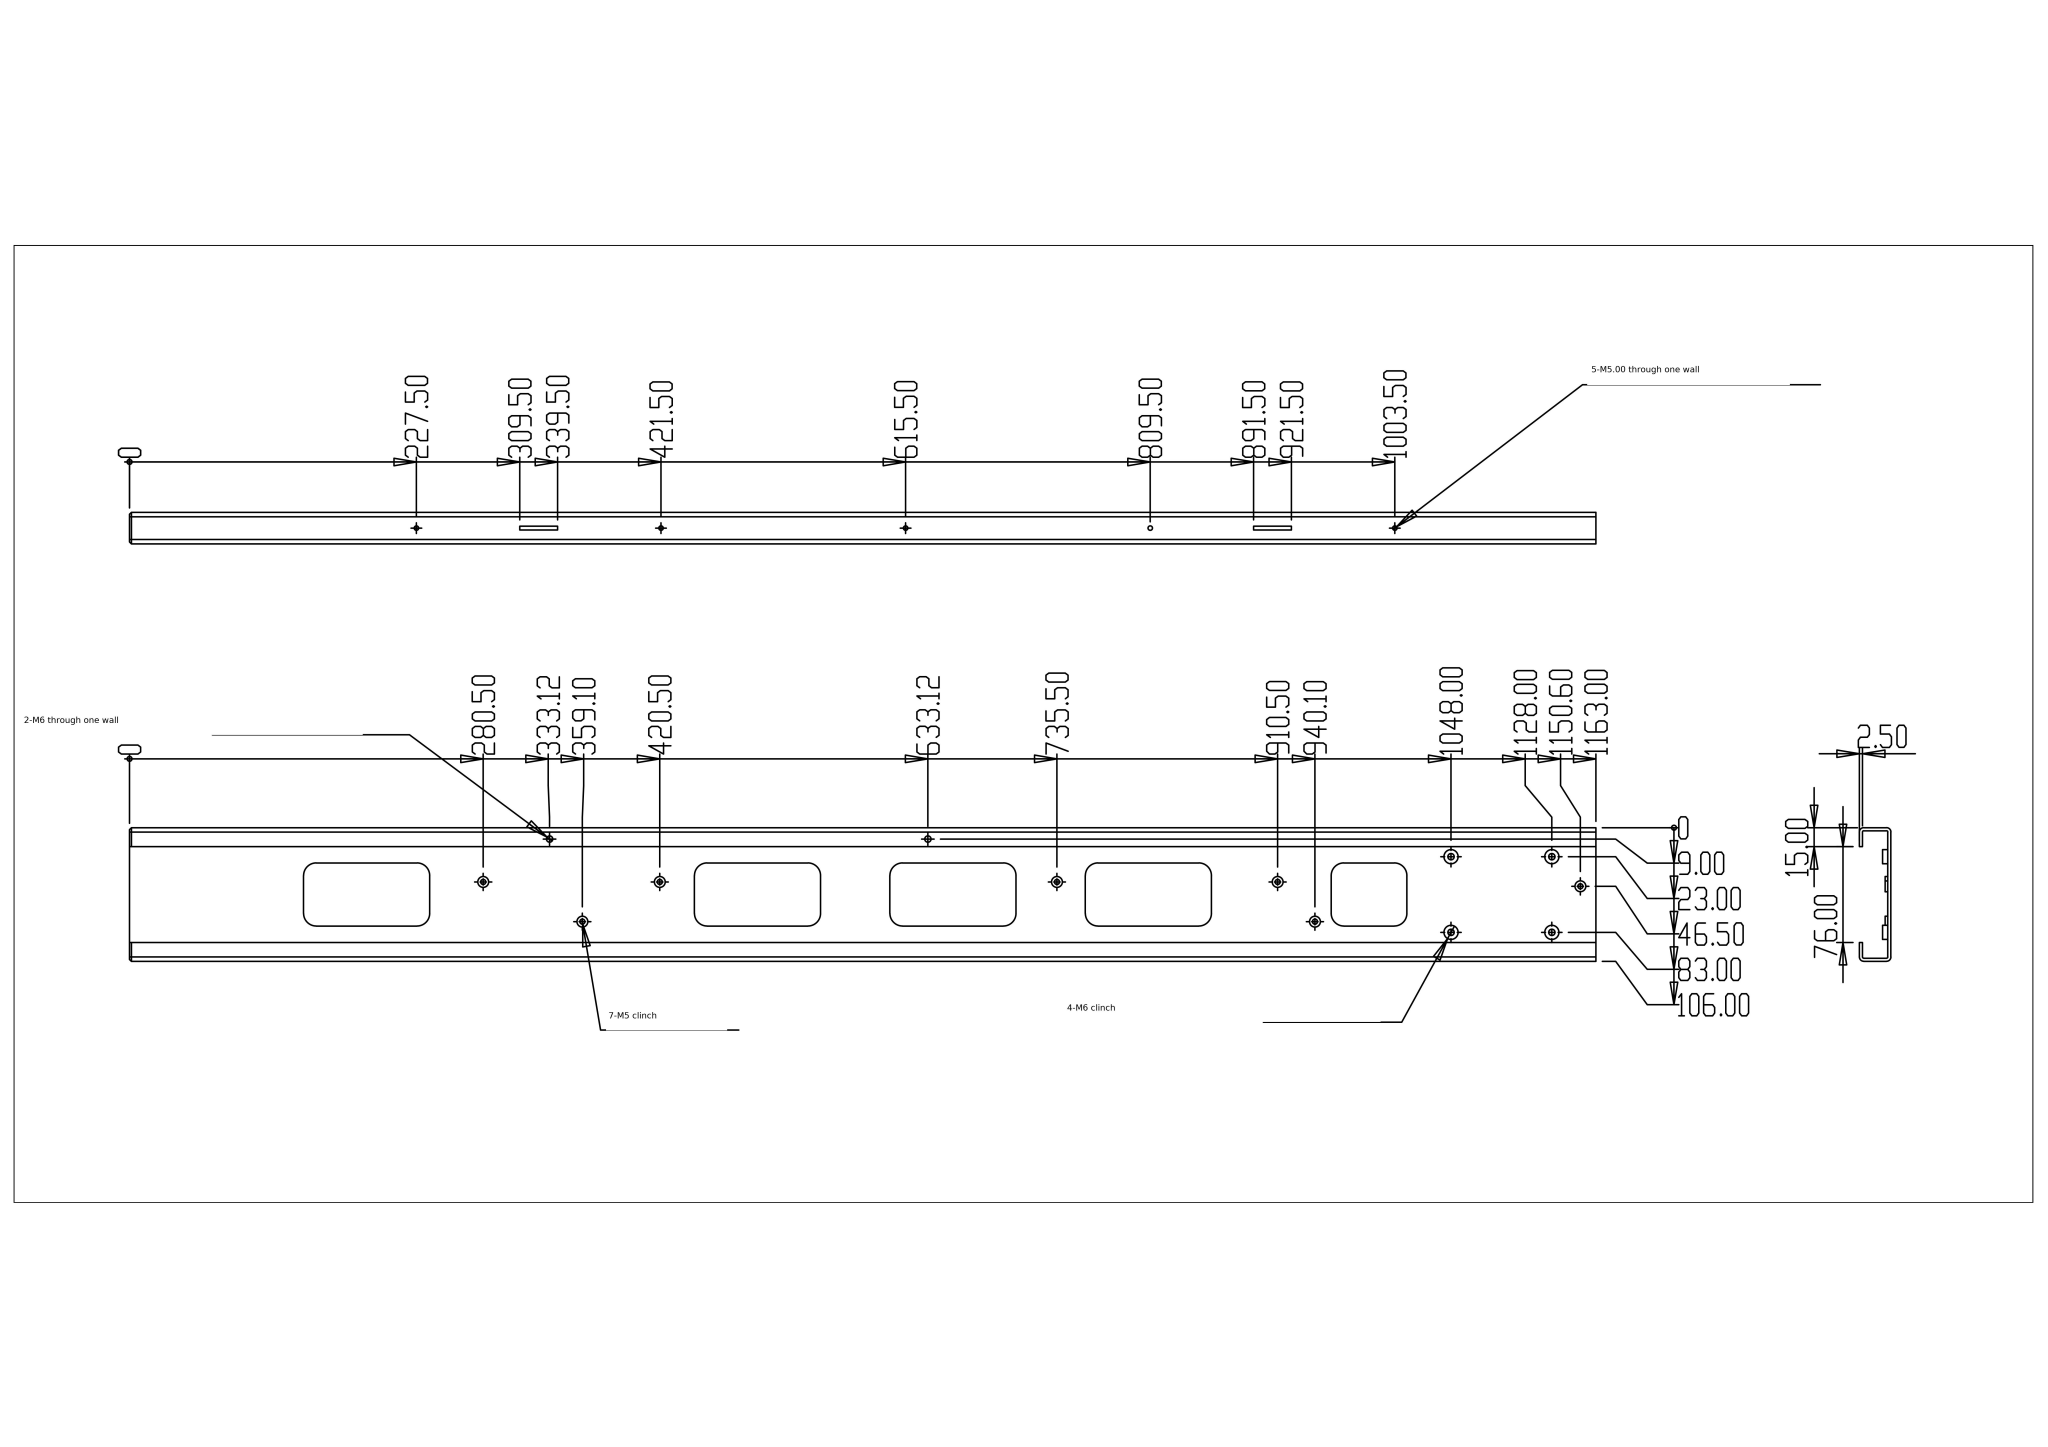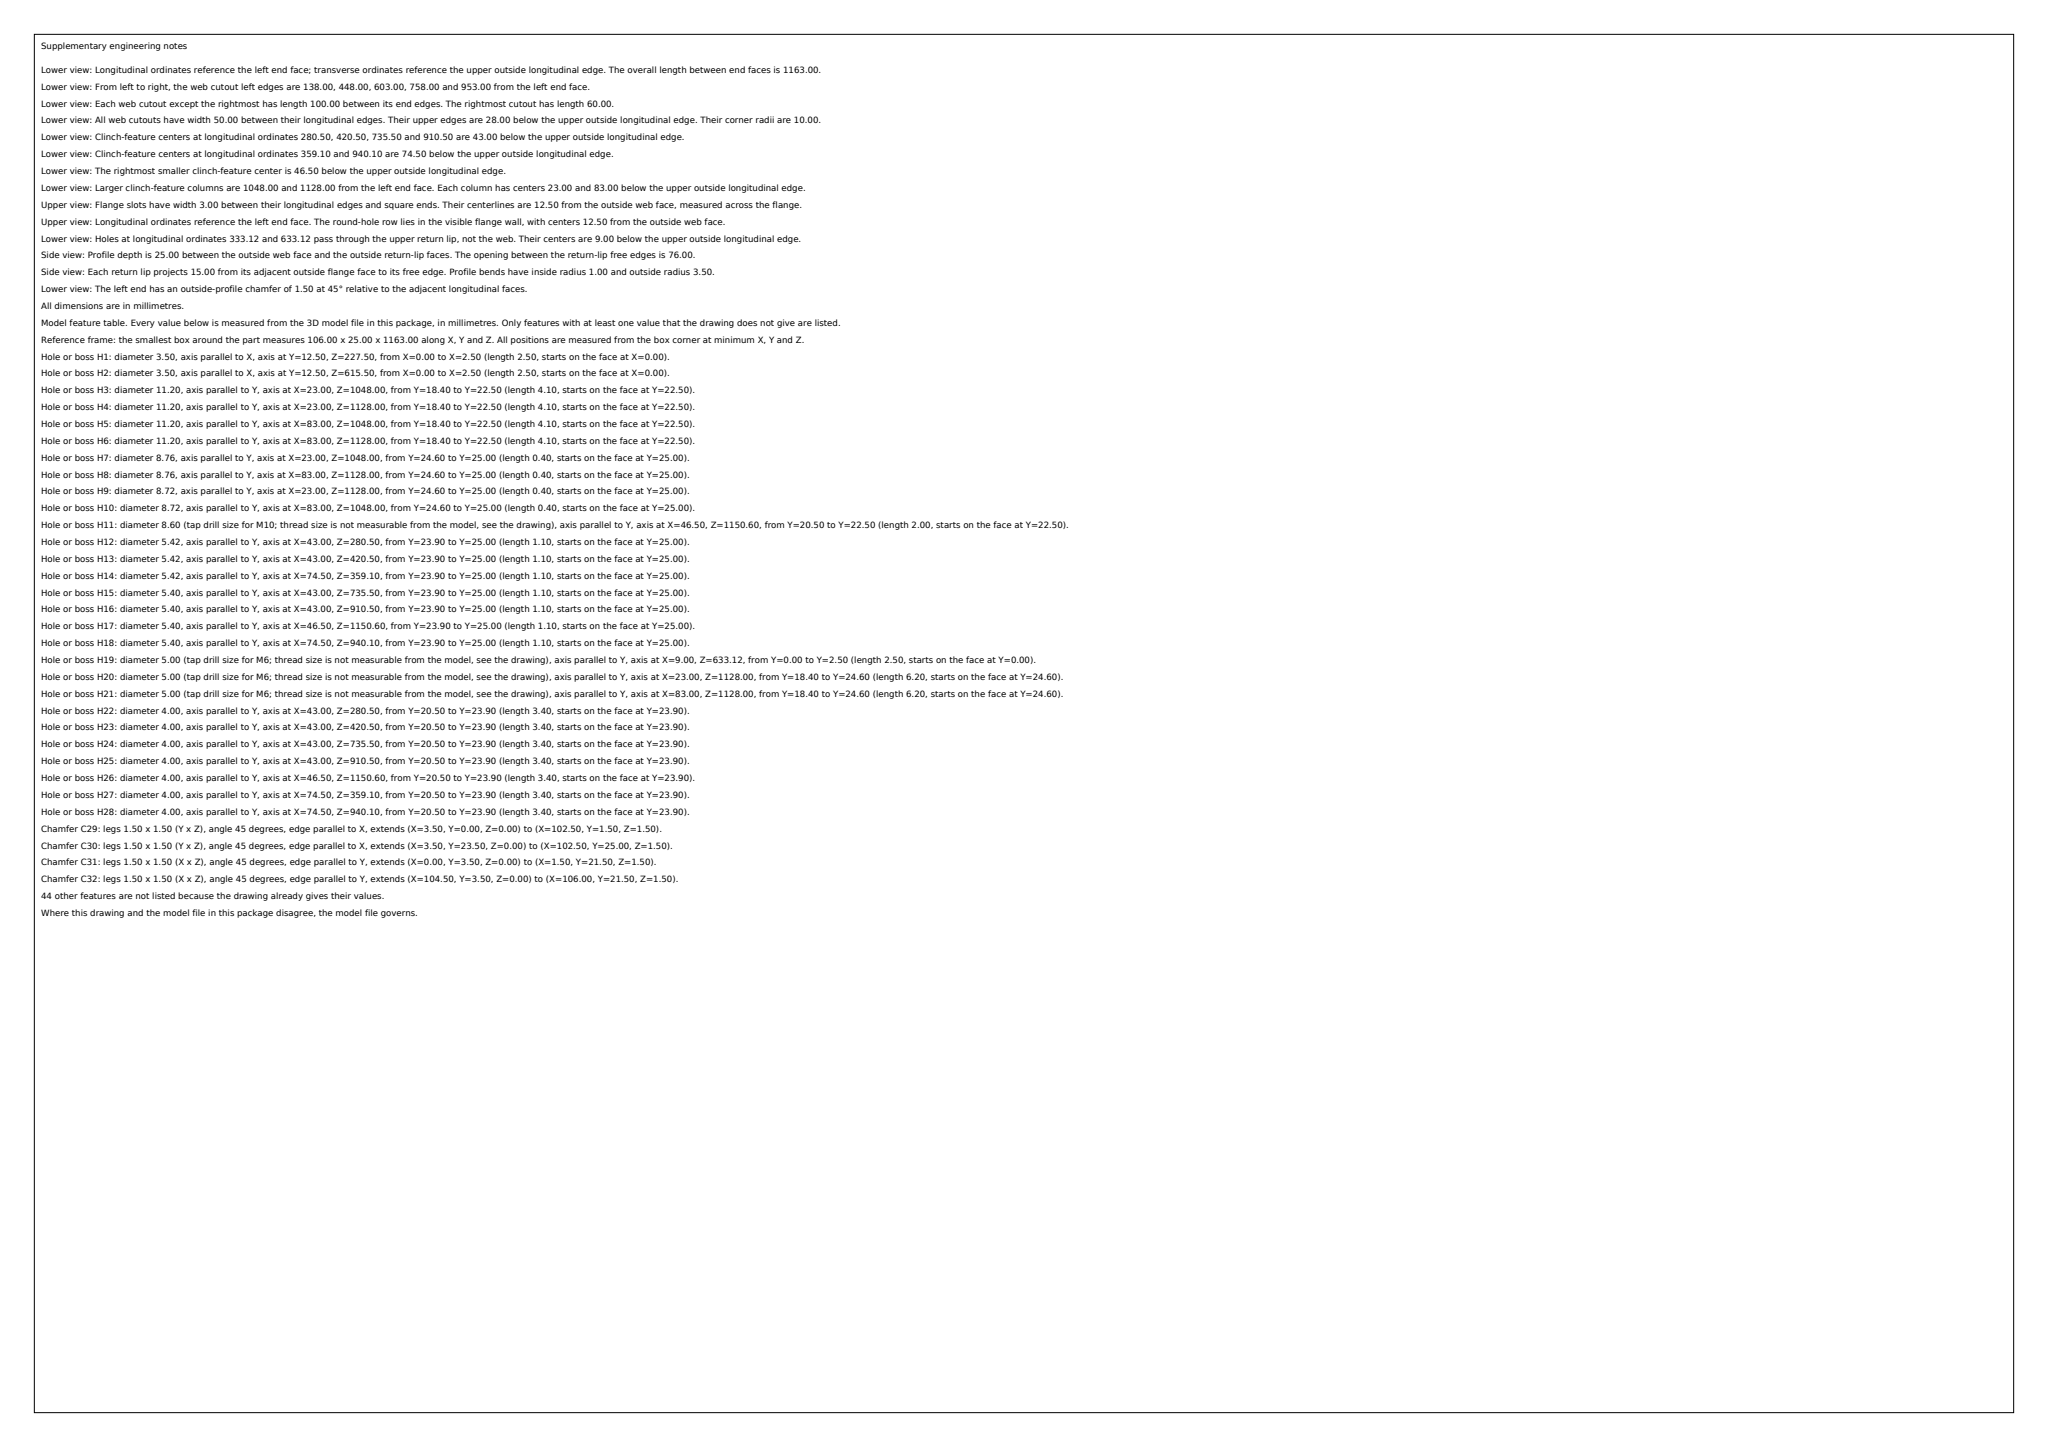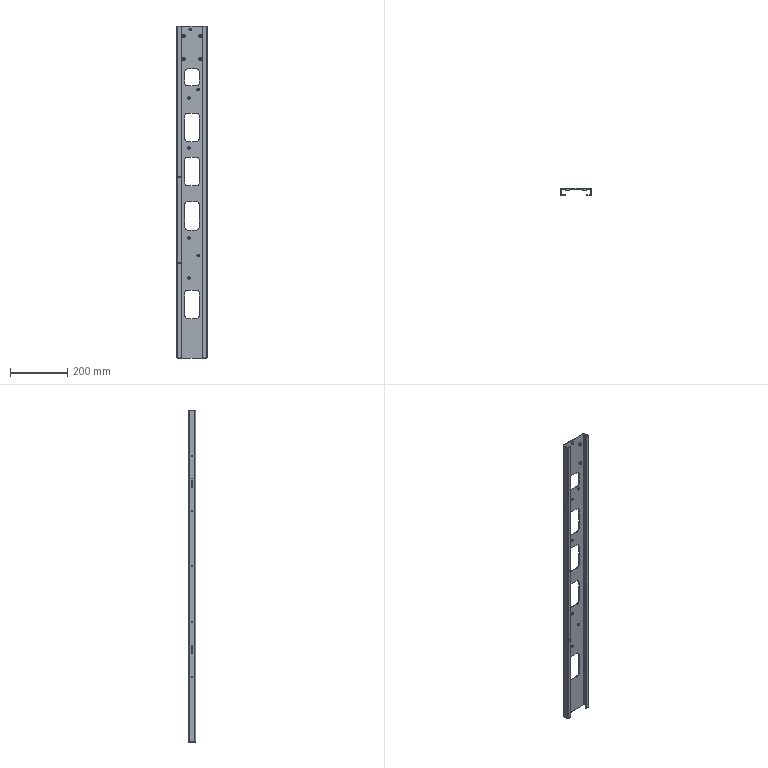Part | SolidWorks | mm | 1 solid | 181 faces | box 106 x 25 x 1163 mm | volume 444564 mm3 | cylinder 108 | plane 69 | cone 4 | commonest cylinder face diameters 20 x20 4 x14 8.6 x14 5.41 x14 5 x12 3.5 x10 11.2 x8 8.75 x4
Drawing notes:
SECTION: OVERALL PROFILE DEPTH 25.00 | from the solid: bbox_xyz y = 25.0; y planes 0.0 and 25.0
ALL ROLL-FORM CORNERS: INNER R1, OUTER R3.5 (4 PL) | from the solid: cylinders Ø2.0 z-axis at (3.5,3.5),(3.5,21.5),(102.5,3.5),(102.5,21.5) L=1163 and Ø7.0 same pos L=1161.5
5 WEB CUTOUTS 50 WIDE x 100 LG (LAST 60 LG), R10 CORNERS | from the solid: x planes 28.0 & 78.0 (5 ea); z pairs 138/238,448/548,603/703,758/858,953/1013; Ø20 y-axis end cyls
WEB CUTOUTS AT Z=138,448,603,758,953; X=28.00 TO 78.00 | from the solid: z planes 138,238,448,548,603,703,758,858,953,1013; x planes 28.0/78.0
7-M5 CLINCH ROWS: X=43.00 (4), X=74.50 (2), X=46.50 (1) | from the solid: Ø4.0 y-axis holes at x=43.0 (z 280.5,420.5,735.5,910.5), x=74.5 (z 359.1,940.1), x=46.5 (z 1150.6)
SIDE WALL SLOTS 30 LG x 3.00 WIDE, Y=11.00 TO 14.00 | from the solid: z planes 309.5/339.5 & 891.5/921.5; y planes 11.0 (2) and 14.0 (2)
5-M5 THRU ONE WALL ON Y=12.50 CL | from the solid: Ø3.5 x-axis holes at y=12.5, z=227.5,421.5,615.5,809.5,1003.5
SIDE HOLES: 4 PL CSK 90° x Ø7.0; HOLE AT 809.50 PLAIN Ø3.5 | from the solid: cones [90.0, 7.0, 4]; five Ø3.5 x-axis holes
build123d program:
from build123d import *

# Parameters (mm, degrees)
BOSS_EXTRUDE1_DEPTH      = 1163
CHAMFER1_SIZE            = 1.5
CUT_EXTRUDE1_REACH       = 1168.823
CUT_EXTRUDE2_REACH       = 1170.088
SKETCH3_R                = 1.75
SKETCH3_W                = 30
SKETCH3_H                = 3
BOSS_EXTRUDE2_DEPTH      = 2
BOSS_EXTRUDE2_DEPTH_BACK = 1.4
SKETCH4_R                = 4.3
SKETCH4_R_2              = 2
BOSS_EXTRUDE3_DEPTH      = 4.1
BOSS_EXTRUDE3_DEPTH_BACK = 2.1
SKETCH5_R                = 5.6
SKETCH5_R_2              = 2.5
CUT_EXTRUDE3_REACH       = 1168.823
SKETCH6_R                = 2.5


with BuildPart() as part:
    # Sketch1 → Boss-Extrude1 (new body)
    with BuildSketch(Plane.XY):
        with BuildLine():
            Line((-76, 0), (-76, 2.5))
            Line((-76, 2.5), (-79, 2.5))
            Line((-79, 2.5), (-87.5, 2.5))
            ThreePointArc((-87.5, 2.5), (-88.207, 2.793), (-88.5, 3.5))
            Line((-88.5, 3.5), (-88.5, 21.5))
            ThreePointArc((-88.5, 21.5), (-88.207, 22.207), (-87.5, 22.5))
            Line((-87.5, 22.5), (11.5, 22.5))
            ThreePointArc((11.5, 22.5), (12.207, 22.207), (12.5, 21.5))
            Line((12.5, 21.5), (12.5, 3.5))
            ThreePointArc((12.5, 3.5), (12.207, 2.793), (11.5, 2.5))
            Line((11.5, 2.5), (3, 2.5))
            Line((3, 2.5), (0, 2.5))
            Line((0, 2.5), (0, 0))
            Line((0, 0), (3, 0))
            Line((3, 0), (11.5, 0))
            ThreePointArc((11.5, 0), (13.975, 1.025), (15, 3.5))
            Line((15, 3.5), (15, 21.5))
            ThreePointArc((15, 21.5), (13.975, 23.975), (11.5, 25))
            Line((11.5, 25), (-87.5, 25))
            ThreePointArc((-87.5, 25), (-89.975, 23.975), (-91, 21.5))
            Line((-91, 21.5), (-91, 3.5))
            ThreePointArc((-91, 3.5), (-89.975, 1.025), (-87.5, 0))
            Line((-87.5, 0), (-79, 0))
            Line((-79, 0), (-76, 0))
        make_face()
    extrude(amount=BOSS_EXTRUDE1_DEPTH)

    # Chamfer1
    chamfer1_edges = [part.edges().sort_by_distance(p)[0] for p in [
        (-81.75, 0, 0),
        (-89.975, 1.025, 0),
        (-91, 12.5, 0),
        (-89.975, 23.975, 0),
        (-38, 25, 0),
        (13.975, 23.975, 0),
        (15, 12.5, 0),
        (13.975, 1.025, 0),
        (5.75, 0, 0),
    ]]
    chamfer(chamfer1_edges, length=CHAMFER1_SIZE)

    # Sketch2 → Cut-Extrude1 (cut, up to next)
    with BuildSketch(Plane(origin=(0, 25, 0), x_dir=(1, 0, 0), z_dir=(0, 1, 0)), mode=Mode.PRIVATE) as cut_extrude1_sk1:
        with BuildLine():
            Line((-23, -953), (-53, -953))
            ThreePointArc((-53, -953), (-60.071, -955.929), (-63, -963))
            Line((-63, -963), (-63, -1003))
            ThreePointArc((-63, -1003), (-60.071, -1010.071), (-53, -1013))
            Line((-53, -1013), (-23, -1013))
            ThreePointArc((-23, -1013), (-15.929, -1010.071), (-13, -1003))
            Line((-13, -1003), (-13, -963))
            ThreePointArc((-13, -963), (-15.929, -955.929), (-23, -953))
        make_face()
    cut_extrude1_tool1 = extrude(cut_extrude1_sk1.sketch, amount=-CUT_EXTRUDE1_REACH, mode=Mode.PRIVATE) & part.part
    # Sketch2 → Cut-Extrude1 (cut, up to next)
    with BuildSketch(Plane(origin=(0, 25, 0), x_dir=(1, 0, 0), z_dir=(0, 1, 0)), mode=Mode.PRIVATE) as cut_extrude1_sk2:
        with BuildLine():
            Line((-23, -603), (-53, -603))
            ThreePointArc((-53, -603), (-60.071, -605.929), (-63, -613))
            Line((-63, -613), (-63, -693))
            ThreePointArc((-63, -693), (-60.071, -700.071), (-53, -703))
            Line((-53, -703), (-23, -703))
            ThreePointArc((-23, -703), (-15.929, -700.071), (-13, -693))
            Line((-13, -693), (-13, -613))
            ThreePointArc((-13, -613), (-15.929, -605.929), (-23, -603))
        make_face()
    cut_extrude1_tool2 = extrude(cut_extrude1_sk2.sketch, amount=-CUT_EXTRUDE1_REACH, mode=Mode.PRIVATE) & part.part
    # Sketch2 → Cut-Extrude1 (cut, up to next)
    with BuildSketch(Plane(origin=(0, 25, 0), x_dir=(1, 0, 0), z_dir=(0, 1, 0)), mode=Mode.PRIVATE) as cut_extrude1_sk3:
        with BuildLine():
            Line((-13, -848), (-13, -768))
            ThreePointArc((-13, -768), (-15.929, -760.929), (-23, -758))
            Line((-23, -758), (-53, -758))
            ThreePointArc((-53, -758), (-60.071, -760.929), (-63, -768))
            Line((-63, -768), (-63, -848))
            ThreePointArc((-63, -848), (-60.071, -855.071), (-53, -858))
            Line((-53, -858), (-23, -858))
            ThreePointArc((-23, -858), (-15.929, -855.071), (-13, -848))
        make_face()
    cut_extrude1_tool3 = extrude(cut_extrude1_sk3.sketch, amount=-CUT_EXTRUDE1_REACH, mode=Mode.PRIVATE) & part.part
    # Sketch2 → Cut-Extrude1 (cut, up to next)
    with BuildSketch(Plane(origin=(0, 25, 0), x_dir=(1, 0, 0), z_dir=(0, 1, 0)), mode=Mode.PRIVATE) as cut_extrude1_sk4:
        with BuildLine():
            Line((-53, -548), (-23, -548))
            ThreePointArc((-23, -548), (-15.929, -545.071), (-13, -538))
            Line((-13, -538), (-13, -458))
            ThreePointArc((-13, -458), (-15.929, -450.929), (-23, -448))
            Line((-23, -448), (-53, -448))
            ThreePointArc((-53, -448), (-60.071, -450.929), (-63, -458))
            Line((-63, -458), (-63, -538))
            ThreePointArc((-63, -538), (-60.071, -545.071), (-53, -548))
        make_face()
    cut_extrude1_tool4 = extrude(cut_extrude1_sk4.sketch, amount=-CUT_EXTRUDE1_REACH, mode=Mode.PRIVATE) & part.part
    # Sketch2 → Cut-Extrude1 (cut, up to next)
    with BuildSketch(Plane(origin=(0, 25, 0), x_dir=(1, 0, 0), z_dir=(0, 1, 0)), mode=Mode.PRIVATE) as cut_extrude1_sk5:
        with BuildLine():
            Line((-13, -228), (-13, -148))
            ThreePointArc((-13, -148), (-15.929, -140.929), (-23, -138))
            Line((-23, -138), (-53, -138))
            ThreePointArc((-53, -138), (-60.071, -140.929), (-63, -148))
            Line((-63, -148), (-63, -228))
            ThreePointArc((-63, -228), (-60.071, -235.071), (-53, -238))
            Line((-53, -238), (-23, -238))
            ThreePointArc((-23, -238), (-15.929, -235.071), (-13, -228))
        make_face()
    cut_extrude1_tool5 = extrude(cut_extrude1_sk5.sketch, amount=-CUT_EXTRUDE1_REACH, mode=Mode.PRIVATE) & part.part
    # Sketch2 → Cut-Extrude1 (cut, up to next)
    with BuildSketch(Plane(origin=(0, 25, 0), x_dir=(1, 0, 0), z_dir=(0, 1, 0)), mode=Mode.PRIVATE) as cut_extrude1_sk6:
        with BuildLine():
            ThreePointArc((-41.795, -1150.6), (-44.5, -1147.895), (-47.205, -1150.6))
            ThreePointArc((-47.205, -1150.6), (-44.5, -1153.305), (-41.795, -1150.6))
        make_face()
    cut_extrude1_tool6 = extrude(cut_extrude1_sk6.sketch, amount=-CUT_EXTRUDE1_REACH, mode=Mode.PRIVATE) & part.part
    # Sketch2 → Cut-Extrude1 (cut, up to next)
    with BuildSketch(Plane(origin=(0, 25, 0), x_dir=(1, 0, 0), z_dir=(0, 1, 0)), mode=Mode.PRIVATE) as cut_extrude1_sk7:
        with BuildLine():
            ThreePointArc((-63.635, -1128), (-68, -1123.635), (-72.365, -1128))
            ThreePointArc((-72.365, -1128), (-68, -1132.365), (-63.635, -1128))
        make_face()
    cut_extrude1_tool7 = extrude(cut_extrude1_sk7.sketch, amount=-CUT_EXTRUDE1_REACH, mode=Mode.PRIVATE) & part.part
    # Sketch2 → Cut-Extrude1 (cut, up to next)
    with BuildSketch(Plane(origin=(0, 25, 0), x_dir=(1, 0, 0), z_dir=(0, 1, 0)), mode=Mode.PRIVATE) as cut_extrude1_sk8:
        with BuildLine():
            ThreePointArc((-3.625, -1128), (-8, -1123.625), (-12.375, -1128))
            ThreePointArc((-12.375, -1128), (-8, -1132.375), (-3.625, -1128))
        make_face()
    cut_extrude1_tool8 = extrude(cut_extrude1_sk8.sketch, amount=-CUT_EXTRUDE1_REACH, mode=Mode.PRIVATE) & part.part
    # Sketch2 → Cut-Extrude1 (cut, up to next)
    with BuildSketch(Plane(origin=(0, 25, 0), x_dir=(1, 0, 0), z_dir=(0, 1, 0)), mode=Mode.PRIVATE) as cut_extrude1_sk9:
        with BuildLine():
            ThreePointArc((-3.635, -1048), (-8, -1043.635), (-12.365, -1048))
            ThreePointArc((-12.365, -1048), (-8, -1052.365), (-3.635, -1048))
        make_face()
    cut_extrude1_tool9 = extrude(cut_extrude1_sk9.sketch, amount=-CUT_EXTRUDE1_REACH, mode=Mode.PRIVATE) & part.part
    # Sketch2 → Cut-Extrude1 (cut, up to next)
    with BuildSketch(Plane(origin=(0, 25, 0), x_dir=(1, 0, 0), z_dir=(0, 1, 0)), mode=Mode.PRIVATE) as cut_extrude1_sk10:
        with BuildLine():
            ThreePointArc((-63.625, -1048), (-68, -1043.625), (-72.375, -1048))
            ThreePointArc((-72.375, -1048), (-68, -1052.375), (-63.625, -1048))
        make_face()
    cut_extrude1_tool10 = extrude(cut_extrude1_sk10.sketch, amount=-CUT_EXTRUDE1_REACH, mode=Mode.PRIVATE) & part.part
    # Sketch2 → Cut-Extrude1 (cut, up to next)
    with BuildSketch(Plane(origin=(0, 25, 0), x_dir=(1, 0, 0), z_dir=(0, 1, 0)), mode=Mode.PRIVATE) as cut_extrude1_sk11:
        with BuildLine():
            ThreePointArc((-50.705, -910.5), (-48, -913.205), (-45.295, -910.5))
            ThreePointArc((-45.295, -910.5), (-48, -907.795), (-50.705, -910.5))
        make_face()
    cut_extrude1_tool11 = extrude(cut_extrude1_sk11.sketch, amount=-CUT_EXTRUDE1_REACH, mode=Mode.PRIVATE) & part.part
    # Sketch2 → Cut-Extrude1 (cut, up to next)
    with BuildSketch(Plane(origin=(0, 25, 0), x_dir=(1, 0, 0), z_dir=(0, 1, 0)), mode=Mode.PRIVATE) as cut_extrude1_sk12:
        with BuildLine():
            ThreePointArc((-19.205, -940.1), (-16.5, -942.805), (-13.795, -940.1))
            ThreePointArc((-13.795, -940.1), (-16.5, -937.395), (-19.205, -940.1))
        make_face()
    cut_extrude1_tool12 = extrude(cut_extrude1_sk12.sketch, amount=-CUT_EXTRUDE1_REACH, mode=Mode.PRIVATE) & part.part
    # Sketch2 → Cut-Extrude1 (cut, up to next)
    with BuildSketch(Plane(origin=(0, 25, 0), x_dir=(1, 0, 0), z_dir=(0, 1, 0)), mode=Mode.PRIVATE) as cut_extrude1_sk13:
        with BuildLine():
            ThreePointArc((-45.295, -735.5), (-48, -732.795), (-50.705, -735.5))
            ThreePointArc((-50.705, -735.5), (-48, -738.205), (-45.295, -735.5))
        make_face()
    cut_extrude1_tool13 = extrude(cut_extrude1_sk13.sketch, amount=-CUT_EXTRUDE1_REACH, mode=Mode.PRIVATE) & part.part
    # Sketch2 → Cut-Extrude1 (cut, up to next)
    with BuildSketch(Plane(origin=(0, 25, 0), x_dir=(1, 0, 0), z_dir=(0, 1, 0)), mode=Mode.PRIVATE) as cut_extrude1_sk14:
        with BuildLine():
            ThreePointArc((-45.295, -420.5), (-48, -417.795), (-50.705, -420.5))
            ThreePointArc((-50.705, -420.5), (-48, -423.205), (-45.295, -420.5))
        make_face()
    cut_extrude1_tool14 = extrude(cut_extrude1_sk14.sketch, amount=-CUT_EXTRUDE1_REACH, mode=Mode.PRIVATE) & part.part
    # Sketch2 → Cut-Extrude1 (cut, up to next)
    with BuildSketch(Plane(origin=(0, 25, 0), x_dir=(1, 0, 0), z_dir=(0, 1, 0)), mode=Mode.PRIVATE) as cut_extrude1_sk15:
        with BuildLine():
            ThreePointArc((-13.795, -359.1), (-16.5, -356.395), (-19.205, -359.1))
            ThreePointArc((-19.205, -359.1), (-16.5, -361.805), (-13.795, -359.1))
        make_face()
    cut_extrude1_tool15 = extrude(cut_extrude1_sk15.sketch, amount=-CUT_EXTRUDE1_REACH, mode=Mode.PRIVATE) & part.part
    # Sketch2 → Cut-Extrude1 (cut, up to next)
    with BuildSketch(Plane(origin=(0, 25, 0), x_dir=(1, 0, 0), z_dir=(0, 1, 0)), mode=Mode.PRIVATE) as cut_extrude1_sk16:
        with BuildLine():
            ThreePointArc((-45.295, -280.5), (-48, -277.795), (-50.705, -280.5))
            ThreePointArc((-50.705, -280.5), (-48, -283.205), (-45.295, -280.5))
        make_face()
    cut_extrude1_tool16 = extrude(cut_extrude1_sk16.sketch, amount=-CUT_EXTRUDE1_REACH, mode=Mode.PRIVATE) & part.part
    add(cut_extrude1_tool1.solids().sort_by_distance((-38, 25, 983))[0], mode=Mode.SUBTRACT)
    add(cut_extrude1_tool2.solids().sort_by_distance((-38, 25, 653))[0], mode=Mode.SUBTRACT)
    add(cut_extrude1_tool3.solids().sort_by_distance((-38, 25, 808))[0], mode=Mode.SUBTRACT)
    add(cut_extrude1_tool4.solids().sort_by_distance((-38, 25, 498))[0], mode=Mode.SUBTRACT)
    add(cut_extrude1_tool5.solids().sort_by_distance((-38, 25, 188))[0], mode=Mode.SUBTRACT)
    add(cut_extrude1_tool6.solids().sort_by_distance((-44.5, 25, 1150.6))[0], mode=Mode.SUBTRACT)
    add(cut_extrude1_tool7.solids().sort_by_distance((-68, 25, 1128))[0], mode=Mode.SUBTRACT)
    add(cut_extrude1_tool8.solids().sort_by_distance((-8, 25, 1128))[0], mode=Mode.SUBTRACT)
    add(cut_extrude1_tool9.solids().sort_by_distance((-8, 25, 1048))[0], mode=Mode.SUBTRACT)
    add(cut_extrude1_tool10.solids().sort_by_distance((-68, 25, 1048))[0], mode=Mode.SUBTRACT)
    add(cut_extrude1_tool11.solids().sort_by_distance((-48, 25, 910.5))[0], mode=Mode.SUBTRACT)
    add(cut_extrude1_tool12.solids().sort_by_distance((-16.5, 25, 940.1))[0], mode=Mode.SUBTRACT)
    add(cut_extrude1_tool13.solids().sort_by_distance((-48, 25, 735.5))[0], mode=Mode.SUBTRACT)
    add(cut_extrude1_tool14.solids().sort_by_distance((-48, 25, 420.5))[0], mode=Mode.SUBTRACT)
    add(cut_extrude1_tool15.solids().sort_by_distance((-16.5, 25, 359.1))[0], mode=Mode.SUBTRACT)
    add(cut_extrude1_tool16.solids().sort_by_distance((-48, 25, 280.5))[0], mode=Mode.SUBTRACT)

    # Sketch3 → Cut-Extrude2 (cut, up to next)
    with BuildSketch(Plane.ZY.offset(91), mode=Mode.PRIVATE) as cut_extrude2_sk1:
        with Locations((421.5, 12.5)):
            Circle(SKETCH3_R)
    cut_extrude2_tool1 = extrude(cut_extrude2_sk1.sketch, amount=-CUT_EXTRUDE2_REACH, mode=Mode.PRIVATE) & part.part
    # Sketch3 → Cut-Extrude2 (cut, up to next)
    with BuildSketch(Plane.ZY.offset(91), mode=Mode.PRIVATE) as cut_extrude2_sk2:
        with Locations((809.5, 12.5)):
            Circle(SKETCH3_R)
    cut_extrude2_tool2 = extrude(cut_extrude2_sk2.sketch, amount=-CUT_EXTRUDE2_REACH, mode=Mode.PRIVATE) & part.part
    # Sketch3 → Cut-Extrude2 (cut, up to next)
    with BuildSketch(Plane.ZY.offset(91), mode=Mode.PRIVATE) as cut_extrude2_sk3:
        with Locations((1003.5, 12.5)):
            Circle(SKETCH3_R)
    cut_extrude2_tool3 = extrude(cut_extrude2_sk3.sketch, amount=-CUT_EXTRUDE2_REACH, mode=Mode.PRIVATE) & part.part
    # Sketch3 → Cut-Extrude2 (cut, up to next)
    with BuildSketch(Plane.ZY.offset(91), mode=Mode.PRIVATE) as cut_extrude2_sk4:
        with Locations((615.5, 12.5)):
            Circle(SKETCH3_R)
    cut_extrude2_tool4 = extrude(cut_extrude2_sk4.sketch, amount=-CUT_EXTRUDE2_REACH, mode=Mode.PRIVATE) & part.part
    # Sketch3 → Cut-Extrude2 (cut, up to next)
    with BuildSketch(Plane.ZY.offset(91), mode=Mode.PRIVATE) as cut_extrude2_sk5:
        with Locations((227.5, 12.5)):
            Circle(SKETCH3_R)
    cut_extrude2_tool5 = extrude(cut_extrude2_sk5.sketch, amount=-CUT_EXTRUDE2_REACH, mode=Mode.PRIVATE) & part.part
    # Sketch3 → Cut-Extrude2 (cut, up to next)
    with BuildSketch(Plane.ZY.offset(91), mode=Mode.PRIVATE) as cut_extrude2_sk6:
        with Locations((324.5, 12.5)):
            Rectangle(SKETCH3_W, SKETCH3_H)
    cut_extrude2_tool6 = extrude(cut_extrude2_sk6.sketch, amount=-CUT_EXTRUDE2_REACH, mode=Mode.PRIVATE) & part.part
    # Sketch3 → Cut-Extrude2 (cut, up to next)
    with BuildSketch(Plane.ZY.offset(91), mode=Mode.PRIVATE) as cut_extrude2_sk7:
        with Locations((906.5, 12.5)):
            Rectangle(SKETCH3_W, SKETCH3_H)
    cut_extrude2_tool7 = extrude(cut_extrude2_sk7.sketch, amount=-CUT_EXTRUDE2_REACH, mode=Mode.PRIVATE) & part.part
    add(cut_extrude2_tool1.solids().sort_by_distance((-91, 12.5, 421.5))[0], mode=Mode.SUBTRACT)
    add(cut_extrude2_tool2.solids().sort_by_distance((-91, 12.5, 809.5))[0], mode=Mode.SUBTRACT)
    add(cut_extrude2_tool3.solids().sort_by_distance((-91, 12.5, 1003.5))[0], mode=Mode.SUBTRACT)
    add(cut_extrude2_tool4.solids().sort_by_distance((-91, 12.5, 615.5))[0], mode=Mode.SUBTRACT)
    add(cut_extrude2_tool5.solids().sort_by_distance((-91, 12.5, 227.5))[0], mode=Mode.SUBTRACT)
    add(cut_extrude2_tool6.solids().sort_by_distance((-91, 12.5, 324.5))[0], mode=Mode.SUBTRACT)
    add(cut_extrude2_tool7.solids().sort_by_distance((-91, 12.5, 906.5))[0], mode=Mode.SUBTRACT)

    # Sketch4 → Boss-Extrude2 (add, two sides: drawn at the far end of the back side and taken through both)
    # profile 1 of 7: a face of its own
    with BuildSketch(Plane.XZ.offset(-22.5).offset(-BOSS_EXTRUDE2_DEPTH_BACK)):
        with Locations(Location((-44.5, 1150.6, 0), (0, 0, 270))):
            Circle(SKETCH4_R)
        with Locations(Location((-44.5, 1150.6, 0), (0, 0, 270))):
            Circle(SKETCH4_R_2, mode=Mode.SUBTRACT)
    # profile 2 of 7: a face of its own
    with BuildSketch(Plane.XZ.offset(-22.5).offset(-BOSS_EXTRUDE2_DEPTH_BACK)):
        with Locations(Location((-48, 910.5, 0), (0, 0, 270))):
            Circle(SKETCH4_R)
        with Locations(Location((-48, 910.5, 0), (0, 0, 270))):
            Circle(SKETCH4_R_2, mode=Mode.SUBTRACT)
    # profile 3 of 7: a face of its own
    with BuildSketch(Plane.XZ.offset(-22.5).offset(-BOSS_EXTRUDE2_DEPTH_BACK)):
        with Locations(Location((-16.5, 940.1, 0), (0, 0, 270))):
            Circle(SKETCH4_R)
        with Locations(Location((-16.5, 940.1, 0), (0, 0, 270))):
            Circle(SKETCH4_R_2, mode=Mode.SUBTRACT)
    # profile 4 of 7: a face of its own
    with BuildSketch(Plane.XZ.offset(-22.5).offset(-BOSS_EXTRUDE2_DEPTH_BACK)):
        with Locations(Location((-48, 735.5, 0), (0, 0, 270))):
            Circle(SKETCH4_R)
        with Locations(Location((-48, 735.5, 0), (0, 0, 270))):
            Circle(SKETCH4_R_2, mode=Mode.SUBTRACT)
    # profile 5 of 7: a face of its own
    with BuildSketch(Plane.XZ.offset(-22.5).offset(-BOSS_EXTRUDE2_DEPTH_BACK)):
        with Locations(Location((-48, 420.5, 0), (0, 0, 270))):
            Circle(SKETCH4_R)
        with Locations(Location((-48, 420.5, 0), (0, 0, 270))):
            Circle(SKETCH4_R_2, mode=Mode.SUBTRACT)
    # profile 6 of 7: a face of its own
    with BuildSketch(Plane.XZ.offset(-22.5).offset(-BOSS_EXTRUDE2_DEPTH_BACK)):
        with Locations(Location((-48, 280.5, 0), (0, 0, 270))):
            Circle(SKETCH4_R)
        with Locations(Location((-48, 280.5, 0), (0, 0, 270))):
            Circle(SKETCH4_R_2, mode=Mode.SUBTRACT)
    # profile 7 of 7: a face of its own
    with BuildSketch(Plane.XZ.offset(-22.5).offset(-BOSS_EXTRUDE2_DEPTH_BACK)):
        with Locations(Location((-16.5, 359.1, 0), (0, 0, 270))):
            Circle(SKETCH4_R)
        with Locations(Location((-16.5, 359.1, 0), (0, 0, 270))):
            Circle(SKETCH4_R_2, mode=Mode.SUBTRACT)
    extrude(amount=BOSS_EXTRUDE2_DEPTH + BOSS_EXTRUDE2_DEPTH_BACK)

    # Sketch5 → Boss-Extrude3 (add, two sides: drawn at the far end of the back side and taken through both)
    # profile 1 of 4: a face of its own
    with BuildSketch(Plane.XZ.offset(-22.5).offset(-BOSS_EXTRUDE3_DEPTH_BACK)):
        with Locations(Location((-68, 1048, 0), (0, 0, 270))):
            Circle(SKETCH5_R)
        with Locations(Location((-68, 1048, 0), (0, 0, 270))):
            Circle(SKETCH5_R_2, mode=Mode.SUBTRACT)
    # profile 2 of 4: a face of its own
    with BuildSketch(Plane.XZ.offset(-22.5).offset(-BOSS_EXTRUDE3_DEPTH_BACK)):
        with Locations(Location((-68, 1128, 0), (0, 0, 270))):
            Circle(SKETCH5_R)
        with Locations(Location((-68, 1128, 0), (0, 0, 270))):
            Circle(SKETCH5_R_2, mode=Mode.SUBTRACT)
    # profile 3 of 4: a face of its own
    with BuildSketch(Plane.XZ.offset(-22.5).offset(-BOSS_EXTRUDE3_DEPTH_BACK)):
        with Locations(Location((-8, 1128, 0), (0, 0, 270))):
            Circle(SKETCH5_R)
        with Locations(Location((-8, 1128, 0), (0, 0, 270))):
            Circle(SKETCH5_R_2, mode=Mode.SUBTRACT)
    # profile 4 of 4: a face of its own
    with BuildSketch(Plane.XZ.offset(-22.5).offset(-BOSS_EXTRUDE3_DEPTH_BACK)):
        with Locations(Location((-8, 1048, 0), (0, 0, 270))):
            Circle(SKETCH5_R)
        with Locations(Location((-8, 1048, 0), (0, 0, 270))):
            Circle(SKETCH5_R_2, mode=Mode.SUBTRACT)
    extrude(amount=BOSS_EXTRUDE3_DEPTH + BOSS_EXTRUDE3_DEPTH_BACK)

    # Sketch6 → Cut-Extrude3 (cut, up to next)
    with BuildSketch(Plane.XZ, mode=Mode.PRIVATE) as cut_extrude3_sk1:
        with Locations(Location((-82, 333.12, 0), (0, 0, 270))):
            Circle(SKETCH6_R)
    cut_extrude3_tool1 = extrude(cut_extrude3_sk1.sketch, amount=-CUT_EXTRUDE3_REACH, mode=Mode.PRIVATE) & part.part
    # Sketch6 → Cut-Extrude3 (cut, up to next)
    with BuildSketch(Plane.XZ, mode=Mode.PRIVATE) as cut_extrude3_sk2:
        with Locations(Location((-82, 633.12, 0), (0, 0, 270))):
            Circle(SKETCH6_R)
    cut_extrude3_tool2 = extrude(cut_extrude3_sk2.sketch, amount=-CUT_EXTRUDE3_REACH, mode=Mode.PRIVATE) & part.part
    add(cut_extrude3_tool1.solids().sort_by_distance((-82, 0, 333.12))[0], mode=Mode.SUBTRACT)
    add(cut_extrude3_tool2.solids().sort_by_distance((-82, 0, 633.12))[0], mode=Mode.SUBTRACT)


solid = part.part